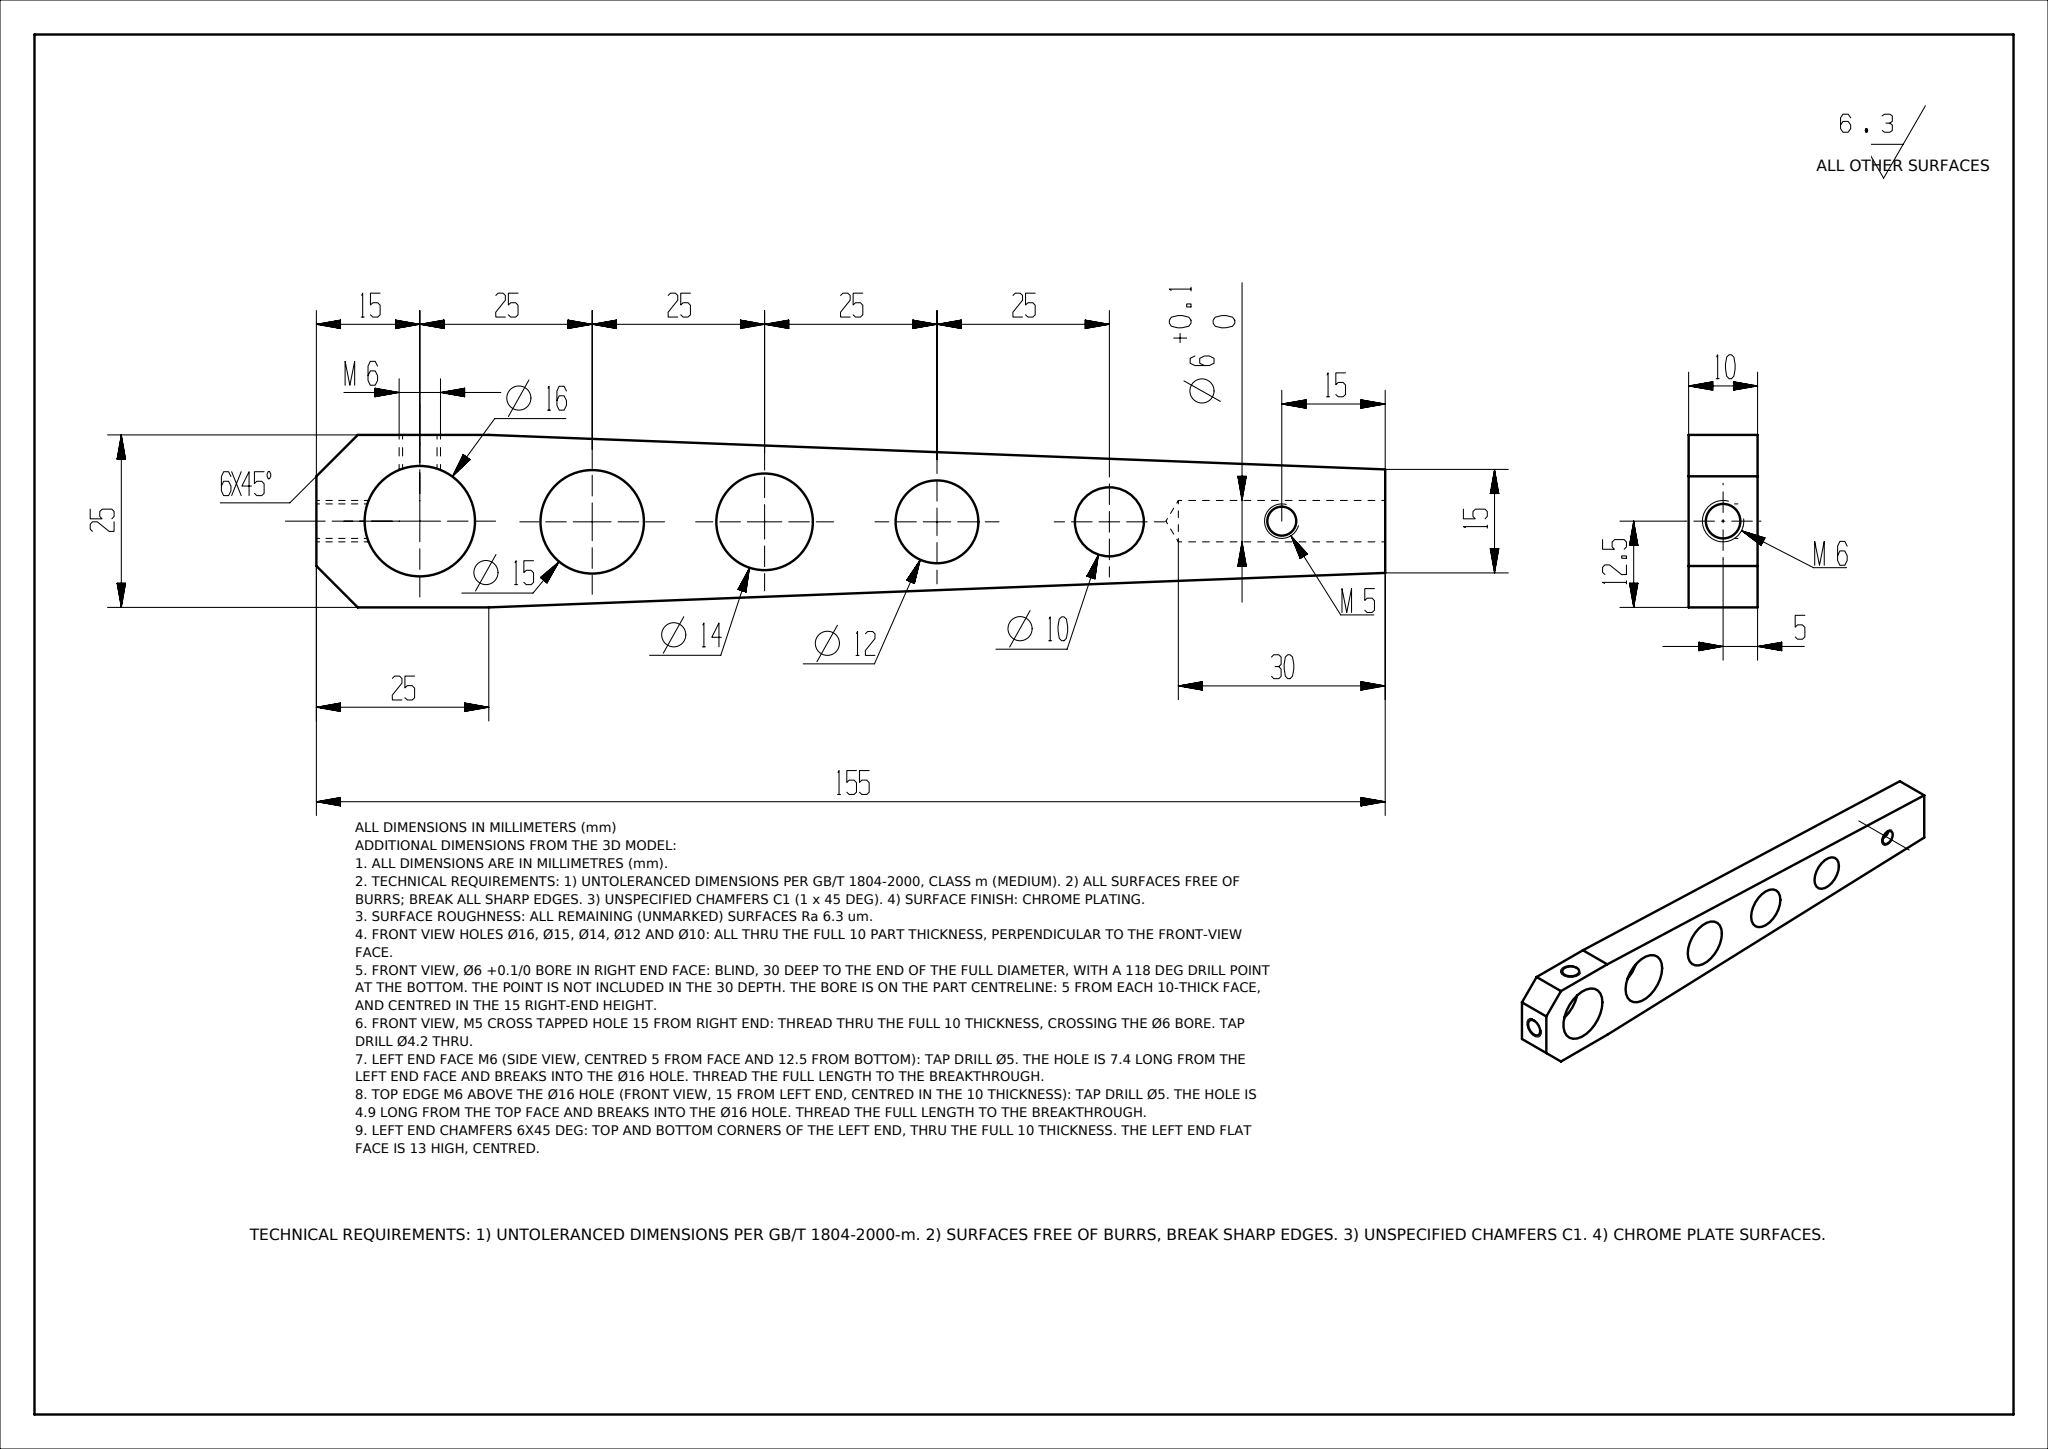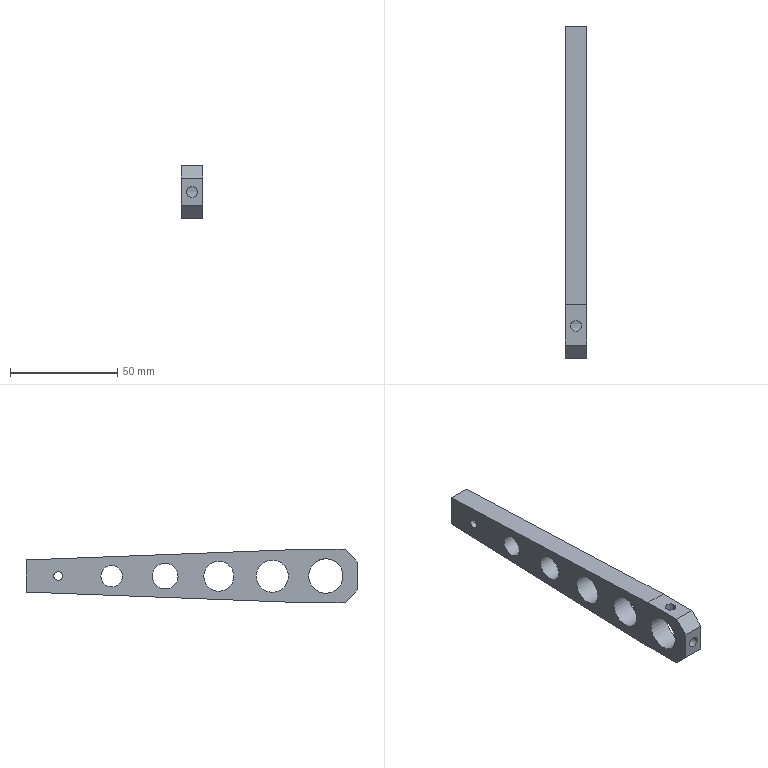Part | NX | mm | 1 solid | 21 faces | box 10 x 155 x 25 mm | volume 23501 mm3 | plane 10 | cylinder 10 | cone 1 | commonest cylinder face diameters 5 x2 4.2 x2 16 x1 15 x1 14 x1 12 x1 10 x1 6 x1
STEP:
#1=CARTESIAN_POINT('',(0.,0.,0.));
#2=DIRECTION('',(0.,0.,1.));
#3=DIRECTION('',(1.,0.,0.));
#4=AXIS2_PLACEMENT_3D('',#1,#2,#3);
#5=(LENGTH_UNIT()NAMED_UNIT(*)SI_UNIT(.MILLI.,.METRE.));
#6=UNCERTAINTY_MEASURE_WITH_UNIT(LENGTH_MEASURE(0.0508),#5,'','');
#7=(NAMED_UNIT(*)PLANE_ANGLE_UNIT()SI_UNIT($,.RADIAN.));
#8=PLANE_ANGLE_MEASURE_WITH_UNIT(PLANE_ANGLE_MEASURE(0.01745),#7);
#9=DIMENSIONAL_EXPONENTS(0.,0.,0.,0.,0.,0.,0.);
#10=(CONVERSION_BASED_UNIT('',#8)NAMED_UNIT(#9)PLANE_ANGLE_UNIT());
#11=(NAMED_UNIT(*)SI_UNIT($,.STERADIAN.)SOLID_ANGLE_UNIT());
#12=(GEOMETRIC_REPRESENTATION_CONTEXT(3)GLOBAL_UNCERTAINTY_ASSIGNED_CONTEXT((#6))GLOBAL_UNIT_ASSIGNED_CONTEXT((#5,#10,#11))REPRESENTATION_CONTEXT('',''));
#13=SHAPE_REPRESENTATION('',(#4),#12);
#14=CARTESIAN_POINT('',(5.,-15.,2.5));
#15=VERTEX_POINT('',#14);
#16=CARTESIAN_POINT('',(5.,-15.,-0.));
#17=DIRECTION('',(0.,1.,-0.));
#18=DIRECTION('',(0.,0.,1.));
#19=AXIS2_PLACEMENT_3D('',#16,#17,#18);
#20=CIRCLE('',#19,2.5);
#21=EDGE_CURVE('',#15,#15,#20,.T.);
#22=ORIENTED_EDGE('',*,*,#21,.T.);
#23=EDGE_LOOP('',(#22));
#24=FACE_BOUND('',#23,.T.);
#25=CARTESIAN_POINT('',(0.,-15.,6.5));
#26=VERTEX_POINT('',#25);
#27=CARTESIAN_POINT('',(0.,-15.,-6.5));
#28=VERTEX_POINT('',#27);
#29=CARTESIAN_POINT('',(0.,-15.,12.5));
#30=DIRECTION('',(0.,-0.,-1.));
#31=VECTOR('',#30,1.);
#32=LINE('',#29,#31);
#33=EDGE_CURVE('',#26,#28,#32,.T.);
#34=ORIENTED_EDGE('',*,*,#33,.T.);
#35=CARTESIAN_POINT('',(10.,-15.,-6.5));
#36=VERTEX_POINT('',#35);
#37=CARTESIAN_POINT('',(10.,-15.,-6.5));
#38=DIRECTION('',(1.,0.,0.));
#39=VECTOR('',#38,1.);
#40=LINE('',#37,#39);
#41=EDGE_CURVE('',#28,#36,#40,.T.);
#42=ORIENTED_EDGE('',*,*,#41,.T.);
#43=CARTESIAN_POINT('',(10.,-15.,6.5));
#44=VERTEX_POINT('',#43);
#45=CARTESIAN_POINT('',(10.,-15.,12.5));
#46=DIRECTION('',(0.,-0.,-1.));
#47=VECTOR('',#46,1.);
#48=LINE('',#45,#47);
#49=EDGE_CURVE('',#44,#36,#48,.T.);
#50=ORIENTED_EDGE('',*,*,#49,.F.);
#51=CARTESIAN_POINT('',(10.,-15.,6.5));
#52=DIRECTION('',(-1.,0.,0.));
#53=VECTOR('',#52,1.);
#54=LINE('',#51,#53);
#55=EDGE_CURVE('',#44,#26,#54,.T.);
#56=ORIENTED_EDGE('',*,*,#55,.T.);
#57=EDGE_LOOP('',(#34,#42,#50,#56));
#58=FACE_BOUND('',#57,.T.);
#59=CARTESIAN_POINT('',(10.,-15.,12.5));
#60=DIRECTION('',(0.,1.,-0.));
#61=DIRECTION('',(0.,0.,1.));
#62=AXIS2_PLACEMENT_3D('',#59,#60,#61);
#63=PLANE('',#62);
#64=ADVANCED_FACE('',(#24,#58),#63,.F.);
#65=CARTESIAN_POINT('',(0.,-9.,-12.5));
#66=VERTEX_POINT('',#65);
#67=CARTESIAN_POINT('',(0.,10.,-12.5));
#68=VERTEX_POINT('',#67);
#69=CARTESIAN_POINT('',(0.,-15.,-12.5));
#70=DIRECTION('',(0.,1.,0.));
#71=VECTOR('',#70,1.);
#72=LINE('',#69,#71);
#73=EDGE_CURVE('',#66,#68,#72,.T.);
#74=ORIENTED_EDGE('',*,*,#73,.T.);
#75=CARTESIAN_POINT('',(10.,10.,-12.5));
#76=VERTEX_POINT('',#75);
#77=CARTESIAN_POINT('',(10.,10.,-12.5));
#78=DIRECTION('',(1.,0.,0.));
#79=VECTOR('',#78,1.);
#80=LINE('',#77,#79);
#81=EDGE_CURVE('',#68,#76,#80,.T.);
#82=ORIENTED_EDGE('',*,*,#81,.T.);
#83=CARTESIAN_POINT('',(10.,-9.,-12.5));
#84=VERTEX_POINT('',#83);
#85=CARTESIAN_POINT('',(10.,-15.,-12.5));
#86=DIRECTION('',(0.,1.,0.));
#87=VECTOR('',#86,1.);
#88=LINE('',#85,#87);
#89=EDGE_CURVE('',#84,#76,#88,.T.);
#90=ORIENTED_EDGE('',*,*,#89,.F.);
#91=CARTESIAN_POINT('',(10.,-9.,-12.5));
#92=DIRECTION('',(-1.,0.,0.));
#93=VECTOR('',#92,1.);
#94=LINE('',#91,#93);
#95=EDGE_CURVE('',#84,#66,#94,.T.);
#96=ORIENTED_EDGE('',*,*,#95,.T.);
#97=EDGE_LOOP('',(#74,#82,#90,#96));
#98=FACE_OUTER_BOUND('',#97,.T.);
#99=CARTESIAN_POINT('',(10.,-15.,-12.5));
#100=DIRECTION('',(0.,-0.,1.));
#101=DIRECTION('',(0.,-1.,-0.));
#102=AXIS2_PLACEMENT_3D('',#99,#100,#101);
#103=PLANE('',#102);
#104=ADVANCED_FACE('',(#98),#103,.F.);
#105=CARTESIAN_POINT('',(5.,140.,-3.));
#106=VERTEX_POINT('',#105);
#107=CARTESIAN_POINT('',(5.,140.,0.));
#108=DIRECTION('',(0.,-1.,0.));
#109=DIRECTION('',(0.,0.,-1.));
#110=AXIS2_PLACEMENT_3D('',#107,#108,#109);
#111=CIRCLE('',#110,3.);
#112=EDGE_CURVE('',#106,#106,#111,.T.);
#113=ORIENTED_EDGE('',*,*,#112,.T.);
#114=EDGE_LOOP('',(#113));
#115=FACE_BOUND('',#114,.T.);
#116=CARTESIAN_POINT('',(10.,140.,-7.5));
#117=VERTEX_POINT('',#116);
#118=CARTESIAN_POINT('',(10.,140.,7.5));
#119=VERTEX_POINT('',#118);
#120=CARTESIAN_POINT('',(10.,140.,-12.5));
#121=DIRECTION('',(0.,0.,1.));
#122=VECTOR('',#121,1.);
#123=LINE('',#120,#122);
#124=EDGE_CURVE('',#117,#119,#123,.T.);
#125=ORIENTED_EDGE('',*,*,#124,.F.);
#126=CARTESIAN_POINT('',(0.,140.,-7.5));
#127=VERTEX_POINT('',#126);
#128=CARTESIAN_POINT('',(10.,140.,-7.5));
#129=DIRECTION('',(-1.,0.,0.));
#130=VECTOR('',#129,1.);
#131=LINE('',#128,#130);
#132=EDGE_CURVE('',#117,#127,#131,.T.);
#133=ORIENTED_EDGE('',*,*,#132,.T.);
#134=CARTESIAN_POINT('',(0.,140.,7.5));
#135=VERTEX_POINT('',#134);
#136=CARTESIAN_POINT('',(0.,140.,-12.5));
#137=DIRECTION('',(0.,0.,1.));
#138=VECTOR('',#137,1.);
#139=LINE('',#136,#138);
#140=EDGE_CURVE('',#127,#135,#139,.T.);
#141=ORIENTED_EDGE('',*,*,#140,.T.);
#142=CARTESIAN_POINT('',(10.,140.,7.5));
#143=DIRECTION('',(1.,0.,0.));
#144=VECTOR('',#143,1.);
#145=LINE('',#142,#144);
#146=EDGE_CURVE('',#135,#119,#145,.T.);
#147=ORIENTED_EDGE('',*,*,#146,.T.);
#148=EDGE_LOOP('',(#125,#133,#141,#147));
#149=FACE_BOUND('',#148,.T.);
#150=CARTESIAN_POINT('',(10.,140.,-12.5));
#151=DIRECTION('',(0.,-1.,0.));
#152=DIRECTION('',(0.,0.,-1.));
#153=AXIS2_PLACEMENT_3D('',#150,#151,#152);
#154=PLANE('',#153);
#155=ADVANCED_FACE('',(#115,#149),#154,.F.);
#156=CARTESIAN_POINT('',(5.,2.5,12.5));
#157=VERTEX_POINT('',#156);
#158=CARTESIAN_POINT('',(5.,0.,12.5));
#159=DIRECTION('',(0.,-0.,-1.));
#160=DIRECTION('',(0.,1.,0.));
#161=AXIS2_PLACEMENT_3D('',#158,#159,#160);
#162=CIRCLE('',#161,2.5);
#163=EDGE_CURVE('',#157,#157,#162,.T.);
#164=ORIENTED_EDGE('',*,*,#163,.T.);
#165=EDGE_LOOP('',(#164));
#166=FACE_BOUND('',#165,.T.);
#167=CARTESIAN_POINT('',(10.,10.,12.5));
#168=VERTEX_POINT('',#167);
#169=CARTESIAN_POINT('',(10.,-9.,12.5));
#170=VERTEX_POINT('',#169);
#171=CARTESIAN_POINT('',(10.,140.,12.5));
#172=DIRECTION('',(0.,-1.,0.));
#173=VECTOR('',#172,1.);
#174=LINE('',#171,#173);
#175=EDGE_CURVE('',#168,#170,#174,.T.);
#176=ORIENTED_EDGE('',*,*,#175,.F.);
#177=CARTESIAN_POINT('',(0.,10.,12.5));
#178=VERTEX_POINT('',#177);
#179=CARTESIAN_POINT('',(10.,10.,12.5));
#180=DIRECTION('',(-1.,0.,0.));
#181=VECTOR('',#180,1.);
#182=LINE('',#179,#181);
#183=EDGE_CURVE('',#168,#178,#182,.T.);
#184=ORIENTED_EDGE('',*,*,#183,.T.);
#185=CARTESIAN_POINT('',(0.,-9.,12.5));
#186=VERTEX_POINT('',#185);
#187=CARTESIAN_POINT('',(0.,140.,12.5));
#188=DIRECTION('',(0.,-1.,0.));
#189=VECTOR('',#188,1.);
#190=LINE('',#187,#189);
#191=EDGE_CURVE('',#178,#186,#190,.T.);
#192=ORIENTED_EDGE('',*,*,#191,.T.);
#193=CARTESIAN_POINT('',(10.,-9.,12.5));
#194=DIRECTION('',(1.,0.,0.));
#195=VECTOR('',#194,1.);
#196=LINE('',#193,#195);
#197=EDGE_CURVE('',#186,#170,#196,.T.);
#198=ORIENTED_EDGE('',*,*,#197,.T.);
#199=EDGE_LOOP('',(#176,#184,#192,#198));
#200=FACE_BOUND('',#199,.T.);
#201=CARTESIAN_POINT('',(10.,140.,12.5));
#202=DIRECTION('',(0.,-0.,-1.));
#203=DIRECTION('',(0.,1.,-0.));
#204=AXIS2_PLACEMENT_3D('',#201,#202,#203);
#205=PLANE('',#204);
#206=ADVANCED_FACE('',(#166,#200),#205,.F.);
#207=CARTESIAN_POINT('',(7.5,0.,8.));
#208=VERTEX_POINT('',#207);
#209=CARTESIAN_POINT('',(7.5,0.,8.));
#210=CARTESIAN_POINT('',(7.5,-0.2725,8.));
#211=CARTESIAN_POINT('',(7.454,-0.5487,7.985));
#212=CARTESIAN_POINT('',(7.367,-0.8054,7.959));
#213=CARTESIAN_POINT('',(7.279,-1.062,7.933));
#214=CARTESIAN_POINT('',(7.149,-1.306,7.896));
#215=CARTESIAN_POINT('',(6.985,-1.52,7.854));
#216=CARTESIAN_POINT('',(6.817,-1.739,7.812));
#217=CARTESIAN_POINT('',(6.61,-1.933,7.765));
#218=CARTESIAN_POINT('',(6.379,-2.085,7.723));
#219=CARTESIAN_POINT('',(6.142,-2.242,7.681));
#220=CARTESIAN_POINT('',(5.874,-2.36,7.644));
#221=CARTESIAN_POINT('',(5.597,-2.428,7.623));
#222=CARTESIAN_POINT('',(5.328,-2.494,7.602));
#223=CARTESIAN_POINT('',(5.042,-2.515,7.594));
#224=CARTESIAN_POINT('',(4.766,-2.489,7.603));
#225=CARTESIAN_POINT('',(4.5,-2.464,7.611));
#226=CARTESIAN_POINT('',(4.236,-2.395,7.634));
#227=CARTESIAN_POINT('',(3.993,-2.288,7.666));
#228=CARTESIAN_POINT('',(3.747,-2.18,7.698));
#229=CARTESIAN_POINT('',(3.516,-2.03,7.74));
#230=CARTESIAN_POINT('',(3.318,-1.85,7.783));
#231=CARTESIAN_POINT('',(3.111,-1.662,7.828));
#232=CARTESIAN_POINT('',(2.934,-1.435,7.874));
#233=CARTESIAN_POINT('',(2.801,-1.188,7.911));
#234=CARTESIAN_POINT('',(2.666,-0.9395,7.949));
#235=CARTESIAN_POINT('',(2.572,-0.6622,7.978));
#236=CARTESIAN_POINT('',(2.529,-0.3805,7.991));
#237=CARTESIAN_POINT('',(2.487,-0.1097,8.004));
#238=CARTESIAN_POINT('',(2.491,0.1728,8.003));
#239=CARTESIAN_POINT('',(2.539,0.4424,7.988));
#240=CARTESIAN_POINT('',(2.587,0.7053,7.973));
#241=CARTESIAN_POINT('',(2.678,0.9631,7.945));
#242=CARTESIAN_POINT('',(2.805,1.196,7.91));
#243=CARTESIAN_POINT('',(2.935,1.435,7.874));
#244=CARTESIAN_POINT('',(3.106,1.654,7.829));
#245=CARTESIAN_POINT('',(3.305,1.837,7.786));
#246=CARTESIAN_POINT('',(3.511,2.028,7.741));
#247=CARTESIAN_POINT('',(3.754,2.186,7.696));
#248=CARTESIAN_POINT('',(4.015,2.298,7.663));
#249=CARTESIAN_POINT('',(4.273,2.409,7.63));
#250=CARTESIAN_POINT('',(4.557,2.477,7.607));
#251=CARTESIAN_POINT('',(4.84,2.495,7.601));
#252=CARTESIAN_POINT('',(5.11,2.512,7.595));
#253=CARTESIAN_POINT('',(5.388,2.484,7.605));
#254=CARTESIAN_POINT('',(5.648,2.414,7.627));
#255=CARTESIAN_POINT('',(5.906,2.345,7.649));
#256=CARTESIAN_POINT('',(6.153,2.234,7.683));
#257=CARTESIAN_POINT('',(6.374,2.088,7.723));
#258=CARTESIAN_POINT('',(6.603,1.938,7.763));
#259=CARTESIAN_POINT('',(6.81,1.747,7.81));
#260=CARTESIAN_POINT('',(6.978,1.53,7.852));
#261=CARTESIAN_POINT('',(7.151,1.306,7.896));
#262=CARTESIAN_POINT('',(7.288,1.047,7.936));
#263=CARTESIAN_POINT('',(7.376,0.7762,7.962));
#264=CARTESIAN_POINT('',(7.458,0.5279,7.986));
#265=CARTESIAN_POINT('',(7.5,0.2623,8.));
#266=CARTESIAN_POINT('',(7.5,0.,8.));
#267=B_SPLINE_CURVE_WITH_KNOTS('',3,(#209,#210,#211,#212,#213,#214,#215,#216,#217,#218,#219,#220,#221,#222,#223,#224,#225,#226,#227,#228,#229,#230,#231,#232,#233,#234,#235,#236,#237,#238,#239,#240,#241,#242,#243,#244,#245,#246,#247,#248,#249,#250,#251,#252,#253,#254,#255,#256,#257,#258,#259,#260,#261,#262,#263,#264,#265,#266),.UNSPECIFIED.,.T.,.F.,(1,3,3,3,3,3,3,3,3,3,3,3,3,3,3,3,3,3,3,3,3,1),(-0.04996,0.,0.05197,0.1038,0.1572,0.2119,0.2649,0.3158,0.3674,0.4214,0.4759,0.5282,0.5792,0.6314,0.6858,0.74,0.7916,0.8425,0.8954,0.95,1.,1.052),.UNSPECIFIED.);
#268=EDGE_CURVE('',#208,#208,#267,.T.);
#269=ORIENTED_EDGE('',*,*,#268,.F.);
#270=EDGE_LOOP('',(#269));
#271=FACE_BOUND('',#270,.T.);
#272=CARTESIAN_POINT('',(5.,-7.599,2.5));
#273=VERTEX_POINT('',#272);
#274=CARTESIAN_POINT('',(5.,-7.599,2.5));
#275=CARTESIAN_POINT('',(5.272,-7.599,2.5));
#276=CARTESIAN_POINT('',(5.548,-7.615,2.454));
#277=CARTESIAN_POINT('',(5.804,-7.642,2.367));
#278=CARTESIAN_POINT('',(6.06,-7.669,2.28));
#279=CARTESIAN_POINT('',(6.304,-7.708,2.15));
#280=CARTESIAN_POINT('',(6.517,-7.749,1.987));
#281=CARTESIAN_POINT('',(6.738,-7.792,1.819));
#282=CARTESIAN_POINT('',(6.931,-7.84,1.611));
#283=CARTESIAN_POINT('',(7.085,-7.88,1.38));
#284=CARTESIAN_POINT('',(7.241,-7.921,1.144));
#285=CARTESIAN_POINT('',(7.359,-7.957,0.8754));
#286=CARTESIAN_POINT('',(7.427,-7.978,0.598));
#287=CARTESIAN_POINT('',(7.494,-7.998,0.3292));
#288=CARTESIAN_POINT('',(7.515,-8.005,0.04411));
#289=CARTESIAN_POINT('',(7.489,-7.997,-0.2321));
#290=CARTESIAN_POINT('',(7.464,-7.989,-0.4989));
#291=CARTESIAN_POINT('',(7.395,-7.967,-0.7646));
#292=CARTESIAN_POINT('',(7.288,-7.936,-1.008));
#293=CARTESIAN_POINT('',(7.179,-7.905,-1.255));
#294=CARTESIAN_POINT('',(7.028,-7.863,-1.486));
#295=CARTESIAN_POINT('',(6.848,-7.821,-1.684));
#296=CARTESIAN_POINT('',(6.66,-7.776,-1.89));
#297=CARTESIAN_POINT('',(6.434,-7.73,-2.067));
#298=CARTESIAN_POINT('',(6.187,-7.692,-2.2));
#299=CARTESIAN_POINT('',(5.938,-7.653,-2.334));
#300=CARTESIAN_POINT('',(5.661,-7.623,-2.428));
#301=CARTESIAN_POINT('',(5.378,-7.609,-2.471));
#302=CARTESIAN_POINT('',(5.108,-7.595,-2.513));
#303=CARTESIAN_POINT('',(4.825,-7.597,-2.509));
#304=CARTESIAN_POINT('',(4.556,-7.612,-2.46));
#305=CARTESIAN_POINT('',(4.294,-7.628,-2.413));
#306=CARTESIAN_POINT('',(4.038,-7.657,-2.322));
#307=CARTESIAN_POINT('',(3.806,-7.693,-2.196));
#308=CARTESIAN_POINT('',(3.567,-7.73,-2.067));
#309=CARTESIAN_POINT('',(3.348,-7.775,-1.896));
#310=CARTESIAN_POINT('',(3.164,-7.818,-1.697));
#311=CARTESIAN_POINT('',(2.973,-7.863,-1.49));
#312=CARTESIAN_POINT('',(2.815,-7.907,-1.247));
#313=CARTESIAN_POINT('',(2.703,-7.939,-0.9862));
#314=CARTESIAN_POINT('',(2.592,-7.971,-0.7276));
#315=CARTESIAN_POINT('',(2.524,-7.993,-0.4446));
#316=CARTESIAN_POINT('',(2.505,-7.998,-0.162));
#317=CARTESIAN_POINT('',(2.488,-8.004,0.1087));
#318=CARTESIAN_POINT('',(2.515,-7.995,0.3865));
#319=CARTESIAN_POINT('',(2.585,-7.974,0.6479));
#320=CARTESIAN_POINT('',(2.655,-7.953,0.906));
#321=CARTESIAN_POINT('',(2.767,-7.919,1.155));
#322=CARTESIAN_POINT('',(2.913,-7.881,1.377));
#323=CARTESIAN_POINT('',(3.064,-7.841,1.606));
#324=CARTESIAN_POINT('',(3.255,-7.794,1.811));
#325=CARTESIAN_POINT('',(3.472,-7.751,1.979));
#326=CARTESIAN_POINT('',(3.696,-7.707,2.152));
#327=CARTESIAN_POINT('',(3.954,-7.666,2.288));
#328=CARTESIAN_POINT('',(4.225,-7.639,2.377));
#329=CARTESIAN_POINT('',(4.473,-7.614,2.458));
#330=CARTESIAN_POINT('',(4.738,-7.599,2.5));
#331=CARTESIAN_POINT('',(5.,-7.599,2.5));
#332=B_SPLINE_CURVE_WITH_KNOTS('',3,(#274,#275,#276,#277,#278,#279,#280,#281,#282,#283,#284,#285,#286,#287,#288,#289,#290,#291,#292,#293,#294,#295,#296,#297,#298,#299,#300,#301,#302,#303,#304,#305,#306,#307,#308,#309,#310,#311,#312,#313,#314,#315,#316,#317,#318,#319,#320,#321,#322,#323,#324,#325,#326,#327,#328,#329,#330,#331),.UNSPECIFIED.,.T.,.F.,(1,3,3,3,3,3,3,3,3,3,3,3,3,3,3,3,3,3,3,3,3,1),(-0.04989,0.,0.0519,0.1037,0.1571,0.2118,0.2648,0.3159,0.3676,0.4215,0.476,0.5283,0.5791,0.6313,0.6858,0.7398,0.7916,0.8426,0.8955,0.9501,1.,1.052),.UNSPECIFIED.);
#333=EDGE_CURVE('',#273,#273,#332,.T.);
#334=ORIENTED_EDGE('',*,*,#333,.F.);
#335=EDGE_LOOP('',(#334));
#336=FACE_BOUND('',#335,.T.);
#337=CARTESIAN_POINT('',(10.,8.,-0.));
#338=VERTEX_POINT('',#337);
#339=CARTESIAN_POINT('',(10.,0.,0.));
#340=DIRECTION('',(1.,0.,0.));
#341=DIRECTION('',(0.,1.,-0.));
#342=AXIS2_PLACEMENT_3D('',#339,#340,#341);
#343=CIRCLE('',#342,8.);
#344=EDGE_CURVE('',#338,#338,#343,.T.);
#345=ORIENTED_EDGE('',*,*,#344,.T.);
#346=EDGE_LOOP('',(#345));
#347=FACE_BOUND('',#346,.T.);
#348=CARTESIAN_POINT('',(0.,8.,-0.));
#349=VERTEX_POINT('',#348);
#350=CARTESIAN_POINT('',(0.,0.,0.));
#351=DIRECTION('',(1.,0.,0.));
#352=DIRECTION('',(0.,1.,-0.));
#353=AXIS2_PLACEMENT_3D('',#350,#351,#352);
#354=CIRCLE('',#353,8.);
#355=EDGE_CURVE('',#349,#349,#354,.T.);
#356=ORIENTED_EDGE('',*,*,#355,.F.);
#357=EDGE_LOOP('',(#356));
#358=FACE_BOUND('',#357,.T.);
#359=CARTESIAN_POINT('',(10.,0.,0.));
#360=DIRECTION('',(-1.,0.,0.));
#361=DIRECTION('',(0.,0.,1.));
#362=AXIS2_PLACEMENT_3D('',#359,#360,#361);
#363=CYLINDRICAL_SURFACE('',#362,8.);
#364=ADVANCED_FACE('',(#271,#336,#347,#358),#363,.F.);
#365=CARTESIAN_POINT('',(10.,125.,2.1));
#366=VERTEX_POINT('',#365);
#367=CARTESIAN_POINT('',(10.,125.,-0.));
#368=DIRECTION('',(-1.,0.,0.));
#369=DIRECTION('',(0.,0.,1.));
#370=AXIS2_PLACEMENT_3D('',#367,#368,#369);
#371=CIRCLE('',#370,2.1);
#372=EDGE_CURVE('',#366,#366,#371,.T.);
#373=ORIENTED_EDGE('',*,*,#372,.T.);
#374=EDGE_LOOP('',(#373));
#375=FACE_BOUND('',#374,.T.);
#376=CARTESIAN_POINT('',(10.,105.,-0.09729));
#377=VERTEX_POINT('',#376);
#378=CARTESIAN_POINT('',(10.,100.,-0.09729));
#379=DIRECTION('',(1.,0.,0.));
#380=DIRECTION('',(0.,1.,-0.));
#381=AXIS2_PLACEMENT_3D('',#378,#379,#380);
#382=CIRCLE('',#381,5.);
#383=EDGE_CURVE('',#377,#377,#382,.T.);
#384=ORIENTED_EDGE('',*,*,#383,.F.);
#385=EDGE_LOOP('',(#384));
#386=FACE_BOUND('',#385,.T.);
#387=CARTESIAN_POINT('',(10.,81.,-0.09729));
#388=VERTEX_POINT('',#387);
#389=CARTESIAN_POINT('',(10.,75.,-0.09729));
#390=DIRECTION('',(1.,0.,0.));
#391=DIRECTION('',(0.,1.,-0.));
#392=AXIS2_PLACEMENT_3D('',#389,#390,#391);
#393=CIRCLE('',#392,6.);
#394=EDGE_CURVE('',#388,#388,#393,.T.);
#395=ORIENTED_EDGE('',*,*,#394,.F.);
#396=EDGE_LOOP('',(#395));
#397=FACE_BOUND('',#396,.T.);
#398=CARTESIAN_POINT('',(10.,57.,-0.09729));
#399=VERTEX_POINT('',#398);
#400=CARTESIAN_POINT('',(10.,50.,-0.09729));
#401=DIRECTION('',(1.,0.,0.));
#402=DIRECTION('',(0.,1.,-0.));
#403=AXIS2_PLACEMENT_3D('',#400,#401,#402);
#404=CIRCLE('',#403,7.);
#405=EDGE_CURVE('',#399,#399,#404,.T.);
#406=ORIENTED_EDGE('',*,*,#405,.F.);
#407=EDGE_LOOP('',(#406));
#408=FACE_BOUND('',#407,.T.);
#409=CARTESIAN_POINT('',(10.,32.5,-0.09729));
#410=VERTEX_POINT('',#409);
#411=CARTESIAN_POINT('',(10.,25.,-0.09729));
#412=DIRECTION('',(1.,0.,0.));
#413=DIRECTION('',(0.,1.,-0.));
#414=AXIS2_PLACEMENT_3D('',#411,#412,#413);
#415=CIRCLE('',#414,7.5);
#416=EDGE_CURVE('',#410,#410,#415,.T.);
#417=ORIENTED_EDGE('',*,*,#416,.F.);
#418=EDGE_LOOP('',(#417));
#419=FACE_BOUND('',#418,.T.);
#420=ORIENTED_EDGE('',*,*,#89,.T.);
#421=CARTESIAN_POINT('',(10.,0.4948,-12.866));
#422=DIRECTION('',(0.,0.9993,0.03843));
#423=VECTOR('',#422,1.);
#424=LINE('',#421,#423);
#425=EDGE_CURVE('',#76,#117,#424,.T.);
#426=ORIENTED_EDGE('',*,*,#425,.T.);
#427=ORIENTED_EDGE('',*,*,#124,.T.);
#428=CARTESIAN_POINT('',(10.,0.4948,12.866));
#429=DIRECTION('',(0.,-0.9993,0.03843));
#430=VECTOR('',#429,1.);
#431=LINE('',#428,#430);
#432=EDGE_CURVE('',#119,#168,#431,.T.);
#433=ORIENTED_EDGE('',*,*,#432,.T.);
#434=ORIENTED_EDGE('',*,*,#175,.T.);
#435=CARTESIAN_POINT('',(10.,-10.75,10.75));
#436=DIRECTION('',(0.,-0.7071,-0.7071));
#437=VECTOR('',#436,1.);
#438=LINE('',#435,#437);
#439=EDGE_CURVE('',#170,#44,#438,.T.);
#440=ORIENTED_EDGE('',*,*,#439,.T.);
#441=ORIENTED_EDGE('',*,*,#49,.T.);
#442=CARTESIAN_POINT('',(10.,-10.75,-10.75));
#443=DIRECTION('',(0.,0.7071,-0.7071));
#444=VECTOR('',#443,1.);
#445=LINE('',#442,#444);
#446=EDGE_CURVE('',#36,#84,#445,.T.);
#447=ORIENTED_EDGE('',*,*,#446,.T.);
#448=EDGE_LOOP('',(#420,#426,#427,#433,#434,#440,#441,#447));
#449=FACE_BOUND('',#448,.T.);
#450=ORIENTED_EDGE('',*,*,#344,.F.);
#451=EDGE_LOOP('',(#450));
#452=FACE_BOUND('',#451,.T.);
#453=CARTESIAN_POINT('',(10.,0.,0.));
#454=DIRECTION('',(1.,0.,0.));
#455=DIRECTION('',(0.,0.,-1.));
#456=AXIS2_PLACEMENT_3D('',#453,#454,#455);
#457=PLANE('',#456);
#458=ADVANCED_FACE('',(#375,#386,#397,#408,#419,#449,#452),#457,.T.);
#459=CARTESIAN_POINT('',(0.,125.,-2.1));
#460=VERTEX_POINT('',#459);
#461=CARTESIAN_POINT('',(0.,125.,-0.));
#462=DIRECTION('',(1.,0.,0.));
#463=DIRECTION('',(0.,0.,-1.));
#464=AXIS2_PLACEMENT_3D('',#461,#462,#463);
#465=CIRCLE('',#464,2.1);
#466=EDGE_CURVE('',#460,#460,#465,.T.);
#467=ORIENTED_EDGE('',*,*,#466,.T.);
#468=EDGE_LOOP('',(#467));
#469=FACE_BOUND('',#468,.T.);
#470=CARTESIAN_POINT('',(0.,105.,-0.09729));
#471=VERTEX_POINT('',#470);
#472=CARTESIAN_POINT('',(0.,100.,-0.09729));
#473=DIRECTION('',(1.,0.,0.));
#474=DIRECTION('',(0.,1.,-0.));
#475=AXIS2_PLACEMENT_3D('',#472,#473,#474);
#476=CIRCLE('',#475,5.);
#477=EDGE_CURVE('',#471,#471,#476,.T.);
#478=ORIENTED_EDGE('',*,*,#477,.T.);
#479=EDGE_LOOP('',(#478));
#480=FACE_BOUND('',#479,.T.);
#481=CARTESIAN_POINT('',(0.,81.,-0.09729));
#482=VERTEX_POINT('',#481);
#483=CARTESIAN_POINT('',(0.,75.,-0.09729));
#484=DIRECTION('',(1.,0.,0.));
#485=DIRECTION('',(0.,1.,-0.));
#486=AXIS2_PLACEMENT_3D('',#483,#484,#485);
#487=CIRCLE('',#486,6.);
#488=EDGE_CURVE('',#482,#482,#487,.T.);
#489=ORIENTED_EDGE('',*,*,#488,.T.);
#490=EDGE_LOOP('',(#489));
#491=FACE_BOUND('',#490,.T.);
#492=CARTESIAN_POINT('',(0.,57.,-0.09729));
#493=VERTEX_POINT('',#492);
#494=CARTESIAN_POINT('',(0.,50.,-0.09729));
#495=DIRECTION('',(1.,0.,0.));
#496=DIRECTION('',(0.,1.,-0.));
#497=AXIS2_PLACEMENT_3D('',#494,#495,#496);
#498=CIRCLE('',#497,7.);
#499=EDGE_CURVE('',#493,#493,#498,.T.);
#500=ORIENTED_EDGE('',*,*,#499,.T.);
#501=EDGE_LOOP('',(#500));
#502=FACE_BOUND('',#501,.T.);
#503=CARTESIAN_POINT('',(0.,32.5,-0.09729));
#504=VERTEX_POINT('',#503);
#505=CARTESIAN_POINT('',(0.,25.,-0.09729));
#506=DIRECTION('',(1.,0.,0.));
#507=DIRECTION('',(0.,1.,-0.));
#508=AXIS2_PLACEMENT_3D('',#505,#506,#507);
#509=CIRCLE('',#508,7.5);
#510=EDGE_CURVE('',#504,#504,#509,.T.);
#511=ORIENTED_EDGE('',*,*,#510,.T.);
#512=EDGE_LOOP('',(#511));
#513=FACE_BOUND('',#512,.T.);
#514=ORIENTED_EDGE('',*,*,#140,.F.);
#515=CARTESIAN_POINT('',(0.,140.,-7.5));
#516=DIRECTION('',(0.,-0.9993,-0.03843));
#517=VECTOR('',#516,1.);
#518=LINE('',#515,#517);
#519=EDGE_CURVE('',#127,#68,#518,.T.);
#520=ORIENTED_EDGE('',*,*,#519,.T.);
#521=ORIENTED_EDGE('',*,*,#73,.F.);
#522=CARTESIAN_POINT('',(0.,-9.,-12.5));
#523=DIRECTION('',(0.,-0.7071,0.7071));
#524=VECTOR('',#523,1.);
#525=LINE('',#522,#524);
#526=EDGE_CURVE('',#66,#28,#525,.T.);
#527=ORIENTED_EDGE('',*,*,#526,.T.);
#528=ORIENTED_EDGE('',*,*,#33,.F.);
#529=CARTESIAN_POINT('',(0.,-15.,6.5));
#530=DIRECTION('',(0.,0.7071,0.7071));
#531=VECTOR('',#530,1.);
#532=LINE('',#529,#531);
#533=EDGE_CURVE('',#26,#186,#532,.T.);
#534=ORIENTED_EDGE('',*,*,#533,.T.);
#535=ORIENTED_EDGE('',*,*,#191,.F.);
#536=CARTESIAN_POINT('',(0.,10.,12.5));
#537=DIRECTION('',(0.,0.9993,-0.03843));
#538=VECTOR('',#537,1.);
#539=LINE('',#536,#538);
#540=EDGE_CURVE('',#178,#135,#539,.T.);
#541=ORIENTED_EDGE('',*,*,#540,.T.);
#542=EDGE_LOOP('',(#514,#520,#521,#527,#528,#534,#535,#541));
#543=FACE_BOUND('',#542,.T.);
#544=ORIENTED_EDGE('',*,*,#355,.T.);
#545=EDGE_LOOP('',(#544));
#546=FACE_BOUND('',#545,.T.);
#547=CARTESIAN_POINT('',(0.,0.,0.));
#548=DIRECTION('',(1.,0.,0.));
#549=DIRECTION('',(0.,0.,-1.));
#550=AXIS2_PLACEMENT_3D('',#547,#548,#549);
#551=PLANE('',#550);
#552=ADVANCED_FACE('',(#469,#480,#491,#502,#513,#543,#546),#551,.F.);
#553=ORIENTED_EDGE('',*,*,#446,.F.);
#554=ORIENTED_EDGE('',*,*,#41,.F.);
#555=ORIENTED_EDGE('',*,*,#526,.F.);
#556=ORIENTED_EDGE('',*,*,#95,.F.);
#557=EDGE_LOOP('',(#553,#554,#555,#556));
#558=FACE_OUTER_BOUND('',#557,.T.);
#559=CARTESIAN_POINT('',(10.,-9.,-12.5));
#560=DIRECTION('',(0.,0.7071,0.7071));
#561=DIRECTION('',(-1.,0.,0.));
#562=AXIS2_PLACEMENT_3D('',#559,#560,#561);
#563=PLANE('',#562);
#564=ADVANCED_FACE('',(#558),#563,.F.);
#565=ORIENTED_EDGE('',*,*,#439,.F.);
#566=ORIENTED_EDGE('',*,*,#197,.F.);
#567=ORIENTED_EDGE('',*,*,#533,.F.);
#568=ORIENTED_EDGE('',*,*,#55,.F.);
#569=EDGE_LOOP('',(#565,#566,#567,#568));
#570=FACE_OUTER_BOUND('',#569,.T.);
#571=CARTESIAN_POINT('',(10.,-15.,6.5));
#572=DIRECTION('',(0.,0.7071,-0.7071));
#573=DIRECTION('',(-1.,0.,0.));
#574=AXIS2_PLACEMENT_3D('',#571,#572,#573);
#575=PLANE('',#574);
#576=ADVANCED_FACE('',(#570),#575,.F.);
#577=ORIENTED_EDGE('',*,*,#432,.F.);
#578=ORIENTED_EDGE('',*,*,#146,.F.);
#579=ORIENTED_EDGE('',*,*,#540,.F.);
#580=ORIENTED_EDGE('',*,*,#183,.F.);
#581=EDGE_LOOP('',(#577,#578,#579,#580));
#582=FACE_OUTER_BOUND('',#581,.T.);
#583=CARTESIAN_POINT('',(10.,10.,12.5));
#584=DIRECTION('',(0.,-0.03843,-0.9993));
#585=DIRECTION('',(-1.,0.,0.));
#586=AXIS2_PLACEMENT_3D('',#583,#584,#585);
#587=PLANE('',#586);
#588=ADVANCED_FACE('',(#582),#587,.F.);
#589=ORIENTED_EDGE('',*,*,#425,.F.);
#590=ORIENTED_EDGE('',*,*,#81,.F.);
#591=ORIENTED_EDGE('',*,*,#519,.F.);
#592=ORIENTED_EDGE('',*,*,#132,.F.);
#593=EDGE_LOOP('',(#589,#590,#591,#592));
#594=FACE_OUTER_BOUND('',#593,.T.);
#595=CARTESIAN_POINT('',(10.,140.,-7.5));
#596=DIRECTION('',(0.,-0.03843,0.9993));
#597=DIRECTION('',(-1.,0.,0.));
#598=AXIS2_PLACEMENT_3D('',#595,#596,#597);
#599=PLANE('',#598);
#600=ADVANCED_FACE('',(#594),#599,.F.);
#601=ORIENTED_EDGE('',*,*,#510,.F.);
#602=EDGE_LOOP('',(#601));
#603=FACE_BOUND('',#602,.T.);
#604=ORIENTED_EDGE('',*,*,#416,.T.);
#605=EDGE_LOOP('',(#604));
#606=FACE_BOUND('',#605,.T.);
#607=CARTESIAN_POINT('',(0.,25.,-0.09729));
#608=DIRECTION('',(1.,0.,0.));
#609=DIRECTION('',(0.,0.,-1.));
#610=AXIS2_PLACEMENT_3D('',#607,#608,#609);
#611=CYLINDRICAL_SURFACE('',#610,7.5);
#612=ADVANCED_FACE('',(#603,#606),#611,.F.);
#613=ORIENTED_EDGE('',*,*,#499,.F.);
#614=EDGE_LOOP('',(#613));
#615=FACE_BOUND('',#614,.T.);
#616=ORIENTED_EDGE('',*,*,#405,.T.);
#617=EDGE_LOOP('',(#616));
#618=FACE_BOUND('',#617,.T.);
#619=CARTESIAN_POINT('',(0.,50.,-0.09729));
#620=DIRECTION('',(1.,0.,0.));
#621=DIRECTION('',(0.,0.,-1.));
#622=AXIS2_PLACEMENT_3D('',#619,#620,#621);
#623=CYLINDRICAL_SURFACE('',#622,7.);
#624=ADVANCED_FACE('',(#615,#618),#623,.F.);
#625=ORIENTED_EDGE('',*,*,#488,.F.);
#626=EDGE_LOOP('',(#625));
#627=FACE_BOUND('',#626,.T.);
#628=ORIENTED_EDGE('',*,*,#394,.T.);
#629=EDGE_LOOP('',(#628));
#630=FACE_BOUND('',#629,.T.);
#631=CARTESIAN_POINT('',(0.,75.,-0.09729));
#632=DIRECTION('',(1.,0.,0.));
#633=DIRECTION('',(0.,0.,-1.));
#634=AXIS2_PLACEMENT_3D('',#631,#632,#633);
#635=CYLINDRICAL_SURFACE('',#634,6.);
#636=ADVANCED_FACE('',(#627,#630),#635,.F.);
#637=ORIENTED_EDGE('',*,*,#477,.F.);
#638=EDGE_LOOP('',(#637));
#639=FACE_BOUND('',#638,.T.);
#640=ORIENTED_EDGE('',*,*,#383,.T.);
#641=EDGE_LOOP('',(#640));
#642=FACE_BOUND('',#641,.T.);
#643=CARTESIAN_POINT('',(0.,100.,-0.09729));
#644=DIRECTION('',(1.,0.,0.));
#645=DIRECTION('',(0.,0.,-1.));
#646=AXIS2_PLACEMENT_3D('',#643,#644,#645);
#647=CYLINDRICAL_SURFACE('',#646,5.);
#648=ADVANCED_FACE('',(#639,#642),#647,.F.);
#649=CARTESIAN_POINT('',(5.,110.,-3.));
#650=VERTEX_POINT('',#649);
#651=CARTESIAN_POINT('',(5.,110.,0.));
#652=DIRECTION('',(0.,1.,0.));
#653=DIRECTION('',(0.,0.,-1.));
#654=AXIS2_PLACEMENT_3D('',#651,#652,#653);
#655=CIRCLE('',#654,3.);
#656=EDGE_CURVE('',#650,#650,#655,.T.);
#657=ORIENTED_EDGE('',*,*,#656,.T.);
#658=EDGE_LOOP('',(#657));
#659=FACE_BOUND('',#658,.T.);
#660=CARTESIAN_POINT('',(5.,108.197,0.));
#661=VERTEX_POINT('',#660);
#662=VERTEX_LOOP('',#661);
#663=FACE_BOUND('',#662,.T.);
#664=CARTESIAN_POINT('',(5.,110.,0.));
#665=DIRECTION('',(0.,1.,0.));
#666=DIRECTION('',(0.,0.,1.));
#667=AXIS2_PLACEMENT_3D('',#664,#665,#666);
#668=CONICAL_SURFACE('',#667,3.,59.);
#669=ADVANCED_FACE('',(#659,#663),#668,.F.);
#670=CARTESIAN_POINT('',(7.142,125.,2.1));
#671=VERTEX_POINT('',#670);
#672=CARTESIAN_POINT('',(7.142,125.,2.1));
#673=CARTESIAN_POINT('',(7.142,124.799,2.1));
#674=CARTESIAN_POINT('',(7.173,124.596,2.07));
#675=CARTESIAN_POINT('',(7.222,124.409,2.015));
#676=CARTESIAN_POINT('',(7.272,124.224,1.961));
#677=CARTESIAN_POINT('',(7.339,124.05,1.882));
#678=CARTESIAN_POINT('',(7.412,123.892,1.784));
#679=CARTESIAN_POINT('',(7.497,123.707,1.669));
#680=CARTESIAN_POINT('',(7.59,123.54,1.526));
#681=CARTESIAN_POINT('',(7.674,123.399,1.359));
#682=CARTESIAN_POINT('',(7.773,123.235,1.166));
#683=CARTESIAN_POINT('',(7.863,123.1,0.9338));
#684=CARTESIAN_POINT('',(7.921,123.014,0.6823));
#685=CARTESIAN_POINT('',(7.964,122.951,0.4986));
#686=CARTESIAN_POINT('',(7.992,122.912,0.2996));
#687=CARTESIAN_POINT('',(7.998,122.902,0.1009));
#688=CARTESIAN_POINT('',(8.005,122.893,-0.09802));
#689=CARTESIAN_POINT('',(7.991,122.913,-0.3018));
#690=CARTESIAN_POINT('',(7.959,122.959,-0.493));
#691=CARTESIAN_POINT('',(7.928,123.004,-0.6801));
#692=CARTESIAN_POINT('',(7.879,123.075,-0.8598));
#693=CARTESIAN_POINT('',(7.82,123.166,-1.022));
#694=CARTESIAN_POINT('',(7.755,123.266,-1.203));
#695=CARTESIAN_POINT('',(7.676,123.393,-1.367));
#696=CARTESIAN_POINT('',(7.594,123.537,-1.507));
#697=CARTESIAN_POINT('',(7.498,123.707,-1.672));
#698=CARTESIAN_POINT('',(7.397,123.907,-1.809));
#699=CARTESIAN_POINT('',(7.314,124.127,-1.91));
#700=CARTESIAN_POINT('',(7.25,124.295,-1.987));
#701=CARTESIAN_POINT('',(7.196,124.481,-2.044));
#702=CARTESIAN_POINT('',(7.167,124.673,-2.074));
#703=CARTESIAN_POINT('',(7.138,124.866,-2.105));
#704=CARTESIAN_POINT('',(7.135,125.071,-2.108));
#705=CARTESIAN_POINT('',(7.159,125.266,-2.083));
#706=CARTESIAN_POINT('',(7.18,125.434,-2.062));
#707=CARTESIAN_POINT('',(7.22,125.598,-2.02));
#708=CARTESIAN_POINT('',(7.27,125.751,-1.961));
#709=CARTESIAN_POINT('',(7.344,125.975,-1.875));
#710=CARTESIAN_POINT('',(7.441,126.18,-1.753));
#711=CARTESIAN_POINT('',(7.536,126.358,-1.602));
#712=CARTESIAN_POINT('',(7.633,126.539,-1.449));
#713=CARTESIAN_POINT('',(7.731,126.696,-1.262));
#714=CARTESIAN_POINT('',(7.81,126.818,-1.051));
#715=CARTESIAN_POINT('',(7.876,126.92,-0.8744));
#716=CARTESIAN_POINT('',(7.93,127.,-0.676));
#717=CARTESIAN_POINT('',(7.963,127.047,-0.4693));
#718=CARTESIAN_POINT('',(7.996,127.094,-0.2616));
#719=CARTESIAN_POINT('',(8.007,127.111,-0.03951));
#720=CARTESIAN_POINT('',(7.995,127.093,0.1749));
#721=CARTESIAN_POINT('',(7.984,127.076,0.3688));
#722=CARTESIAN_POINT('',(7.953,127.032,0.5614));
#723=CARTESIAN_POINT('',(7.908,126.966,0.7389));
#724=CARTESIAN_POINT('',(7.861,126.897,0.9228));
#725=CARTESIAN_POINT('',(7.798,126.802,1.095));
#726=CARTESIAN_POINT('',(7.728,126.689,1.247));
#727=CARTESIAN_POINT('',(7.648,126.559,1.424));
#728=CARTESIAN_POINT('',(7.556,126.402,1.578));
#729=CARTESIAN_POINT('',(7.468,126.226,1.705));
#730=CARTESIAN_POINT('',(7.368,126.023,1.851));
#731=CARTESIAN_POINT('',(7.269,125.787,1.965));
#732=CARTESIAN_POINT('',(7.208,125.533,2.031));
#733=CARTESIAN_POINT('',(7.167,125.363,2.076));
#734=CARTESIAN_POINT('',(7.142,125.18,2.1));
#735=CARTESIAN_POINT('',(7.142,125.,2.1));
#736=B_SPLINE_CURVE_WITH_KNOTS('',3,(#672,#673,#674,#675,#676,#677,#678,#679,#680,#681,#682,#683,#684,#685,#686,#687,#688,#689,#690,#691,#692,#693,#694,#695,#696,#697,#698,#699,#700,#701,#702,#703,#704,#705,#706,#707,#708,#709,#710,#711,#712,#713,#714,#715,#716,#717,#718,#719,#720,#721,#722,#723,#724,#725,#726,#727,#728,#729,#730,#731,#732,#733,#734,#735),.UNSPECIFIED.,.T.,.F.,(1,3,3,3,3,3,3,3,3,3,3,3,3,3,3,3,3,3,3,3,3,3,3,1),(-0.03946,0.,0.04422,0.08784,0.1392,0.1994,0.2431,0.2868,0.3295,0.3771,0.4332,0.4763,0.5198,0.5571,0.6123,0.6686,0.7157,0.7631,0.8058,0.8499,0.9011,0.9605,1.,1.044),.UNSPECIFIED.);
#737=EDGE_CURVE('',#671,#671,#736,.T.);
#738=ORIENTED_EDGE('',*,*,#737,.T.);
#739=EDGE_LOOP('',(#738));
#740=FACE_BOUND('',#739,.T.);
#741=CARTESIAN_POINT('',(2.858,125.,2.1));
#742=VERTEX_POINT('',#741);
#743=CARTESIAN_POINT('',(2.858,125.,2.1));
#744=CARTESIAN_POINT('',(2.858,125.201,2.1));
#745=CARTESIAN_POINT('',(2.827,125.404,2.07));
#746=CARTESIAN_POINT('',(2.778,125.591,2.015));
#747=CARTESIAN_POINT('',(2.728,125.776,1.961));
#748=CARTESIAN_POINT('',(2.661,125.95,1.882));
#749=CARTESIAN_POINT('',(2.588,126.108,1.784));
#750=CARTESIAN_POINT('',(2.503,126.293,1.669));
#751=CARTESIAN_POINT('',(2.41,126.46,1.526));
#752=CARTESIAN_POINT('',(2.326,126.601,1.359));
#753=CARTESIAN_POINT('',(2.227,126.765,1.166));
#754=CARTESIAN_POINT('',(2.137,126.9,0.9338));
#755=CARTESIAN_POINT('',(2.079,126.986,0.6823));
#756=CARTESIAN_POINT('',(2.036,127.049,0.4986));
#757=CARTESIAN_POINT('',(2.008,127.088,0.2996));
#758=CARTESIAN_POINT('',(2.002,127.098,0.1009));
#759=CARTESIAN_POINT('',(1.995,127.107,-0.09802));
#760=CARTESIAN_POINT('',(2.009,127.087,-0.3018));
#761=CARTESIAN_POINT('',(2.041,127.041,-0.493));
#762=CARTESIAN_POINT('',(2.072,126.996,-0.6801));
#763=CARTESIAN_POINT('',(2.121,126.925,-0.8598));
#764=CARTESIAN_POINT('',(2.18,126.834,-1.022));
#765=CARTESIAN_POINT('',(2.245,126.734,-1.203));
#766=CARTESIAN_POINT('',(2.324,126.607,-1.367));
#767=CARTESIAN_POINT('',(2.406,126.463,-1.507));
#768=CARTESIAN_POINT('',(2.502,126.293,-1.672));
#769=CARTESIAN_POINT('',(2.603,126.093,-1.809));
#770=CARTESIAN_POINT('',(2.686,125.873,-1.91));
#771=CARTESIAN_POINT('',(2.75,125.705,-1.987));
#772=CARTESIAN_POINT('',(2.804,125.519,-2.044));
#773=CARTESIAN_POINT('',(2.833,125.327,-2.074));
#774=CARTESIAN_POINT('',(2.862,125.134,-2.105));
#775=CARTESIAN_POINT('',(2.865,124.929,-2.108));
#776=CARTESIAN_POINT('',(2.841,124.734,-2.083));
#777=CARTESIAN_POINT('',(2.82,124.566,-2.062));
#778=CARTESIAN_POINT('',(2.78,124.402,-2.02));
#779=CARTESIAN_POINT('',(2.73,124.249,-1.961));
#780=CARTESIAN_POINT('',(2.656,124.025,-1.875));
#781=CARTESIAN_POINT('',(2.559,123.82,-1.753));
#782=CARTESIAN_POINT('',(2.464,123.642,-1.602));
#783=CARTESIAN_POINT('',(2.367,123.461,-1.449));
#784=CARTESIAN_POINT('',(2.269,123.304,-1.262));
#785=CARTESIAN_POINT('',(2.19,123.182,-1.051));
#786=CARTESIAN_POINT('',(2.124,123.08,-0.8744));
#787=CARTESIAN_POINT('',(2.07,123.,-0.676));
#788=CARTESIAN_POINT('',(2.037,122.953,-0.4693));
#789=CARTESIAN_POINT('',(2.004,122.906,-0.2616));
#790=CARTESIAN_POINT('',(1.993,122.889,-0.03951));
#791=CARTESIAN_POINT('',(2.005,122.907,0.1749));
#792=CARTESIAN_POINT('',(2.016,122.924,0.3688));
#793=CARTESIAN_POINT('',(2.047,122.968,0.5614));
#794=CARTESIAN_POINT('',(2.092,123.034,0.7389));
#795=CARTESIAN_POINT('',(2.139,123.103,0.9228));
#796=CARTESIAN_POINT('',(2.202,123.198,1.095));
#797=CARTESIAN_POINT('',(2.272,123.311,1.247));
#798=CARTESIAN_POINT('',(2.352,123.441,1.424));
#799=CARTESIAN_POINT('',(2.444,123.598,1.578));
#800=CARTESIAN_POINT('',(2.532,123.774,1.705));
#801=CARTESIAN_POINT('',(2.632,123.977,1.851));
#802=CARTESIAN_POINT('',(2.731,124.213,1.965));
#803=CARTESIAN_POINT('',(2.792,124.467,2.031));
#804=CARTESIAN_POINT('',(2.833,124.637,2.076));
#805=CARTESIAN_POINT('',(2.858,124.82,2.1));
#806=CARTESIAN_POINT('',(2.858,125.,2.1));
#807=B_SPLINE_CURVE_WITH_KNOTS('',3,(#743,#744,#745,#746,#747,#748,#749,#750,#751,#752,#753,#754,#755,#756,#757,#758,#759,#760,#761,#762,#763,#764,#765,#766,#767,#768,#769,#770,#771,#772,#773,#774,#775,#776,#777,#778,#779,#780,#781,#782,#783,#784,#785,#786,#787,#788,#789,#790,#791,#792,#793,#794,#795,#796,#797,#798,#799,#800,#801,#802,#803,#804,#805,#806),.UNSPECIFIED.,.T.,.F.,(1,3,3,3,3,3,3,3,3,3,3,3,3,3,3,3,3,3,3,3,3,3,3,1),(-0.03946,0.,0.04422,0.08784,0.1392,0.1994,0.2431,0.2868,0.3295,0.3771,0.4332,0.4763,0.5198,0.5571,0.6123,0.6686,0.7157,0.7631,0.8058,0.8499,0.9011,0.9605,1.,1.044),.UNSPECIFIED.);
#808=EDGE_CURVE('',#742,#742,#807,.T.);
#809=ORIENTED_EDGE('',*,*,#808,.T.);
#810=EDGE_LOOP('',(#809));
#811=FACE_BOUND('',#810,.T.);
#812=ORIENTED_EDGE('',*,*,#656,.F.);
#813=EDGE_LOOP('',(#812));
#814=FACE_BOUND('',#813,.T.);
#815=ORIENTED_EDGE('',*,*,#112,.F.);
#816=EDGE_LOOP('',(#815));
#817=FACE_BOUND('',#816,.T.);
#818=CARTESIAN_POINT('',(5.,140.,0.));
#819=DIRECTION('',(0.,-1.,0.));
#820=DIRECTION('',(0.,0.,-1.));
#821=AXIS2_PLACEMENT_3D('',#818,#819,#820);
#822=CYLINDRICAL_SURFACE('',#821,3.);
#823=ADVANCED_FACE('',(#740,#811,#814,#817),#822,.F.);
#824=ORIENTED_EDGE('',*,*,#333,.T.);
#825=EDGE_LOOP('',(#824));
#826=FACE_BOUND('',#825,.T.);
#827=ORIENTED_EDGE('',*,*,#21,.F.);
#828=EDGE_LOOP('',(#827));
#829=FACE_BOUND('',#828,.T.);
#830=CARTESIAN_POINT('',(5.,-15.,-0.));
#831=DIRECTION('',(0.,1.,-0.));
#832=DIRECTION('',(0.,0.,1.));
#833=AXIS2_PLACEMENT_3D('',#830,#831,#832);
#834=CYLINDRICAL_SURFACE('',#833,2.5);
#835=ADVANCED_FACE('',(#826,#829),#834,.F.);
#836=ORIENTED_EDGE('',*,*,#268,.T.);
#837=EDGE_LOOP('',(#836));
#838=FACE_BOUND('',#837,.T.);
#839=ORIENTED_EDGE('',*,*,#163,.F.);
#840=EDGE_LOOP('',(#839));
#841=FACE_BOUND('',#840,.T.);
#842=CARTESIAN_POINT('',(5.,0.,12.5));
#843=DIRECTION('',(0.,-0.,-1.));
#844=DIRECTION('',(0.,1.,0.));
#845=AXIS2_PLACEMENT_3D('',#842,#843,#844);
#846=CYLINDRICAL_SURFACE('',#845,2.5);
#847=ADVANCED_FACE('',(#838,#841),#846,.F.);
#848=ORIENTED_EDGE('',*,*,#808,.F.);
#849=EDGE_LOOP('',(#848));
#850=FACE_BOUND('',#849,.T.);
#851=ORIENTED_EDGE('',*,*,#466,.F.);
#852=EDGE_LOOP('',(#851));
#853=FACE_BOUND('',#852,.T.);
#854=CARTESIAN_POINT('',(10.,125.,-0.));
#855=DIRECTION('',(-1.,0.,0.));
#856=DIRECTION('',(0.,0.,1.));
#857=AXIS2_PLACEMENT_3D('',#854,#855,#856);
#858=CYLINDRICAL_SURFACE('',#857,2.1);
#859=ADVANCED_FACE('',(#850,#853),#858,.F.);
#860=ORIENTED_EDGE('',*,*,#372,.F.);
#861=EDGE_LOOP('',(#860));
#862=FACE_BOUND('',#861,.T.);
#863=ORIENTED_EDGE('',*,*,#737,.F.);
#864=EDGE_LOOP('',(#863));
#865=FACE_BOUND('',#864,.T.);
#866=CARTESIAN_POINT('',(10.,125.,-0.));
#867=DIRECTION('',(-1.,0.,0.));
#868=DIRECTION('',(0.,0.,1.));
#869=AXIS2_PLACEMENT_3D('',#866,#867,#868);
#870=CYLINDRICAL_SURFACE('',#869,2.1);
#871=ADVANCED_FACE('',(#862,#865),#870,.F.);
#872=CLOSED_SHELL('',(#64,#104,#155,#206,#364,#458,#552,#564,#576,#588,#600,#612,#624,#636,#648,#669,#823,#835,#847,#859,#871));
#873=MANIFOLD_SOLID_BREP('',#872);
#874=ADVANCED_BREP_SHAPE_REPRESENTATION('',(#873),#12);
#875=SHAPE_REPRESENTATION_RELATIONSHIP('','',#13,#874);
#876=PRESENTATION_LAYER_ASSIGNMENT('','',(#873));
#877=COLOUR_RGB('',0.6941,0.6941,0.6941);
#878=FILL_AREA_STYLE_COLOUR('',#877);
#879=FILL_AREA_STYLE('',(#878));
#880=SURFACE_STYLE_FILL_AREA(#879);
#881=SURFACE_SIDE_STYLE('',(#880));
#882=SURFACE_STYLE_USAGE(.BOTH.,#881);
#883=PRESENTATION_STYLE_ASSIGNMENT((#882));
#884=STYLED_ITEM('',(#883),#873);
#885=MECHANICAL_DESIGN_GEOMETRIC_PRESENTATION_REPRESENTATION('',(#884),#12);